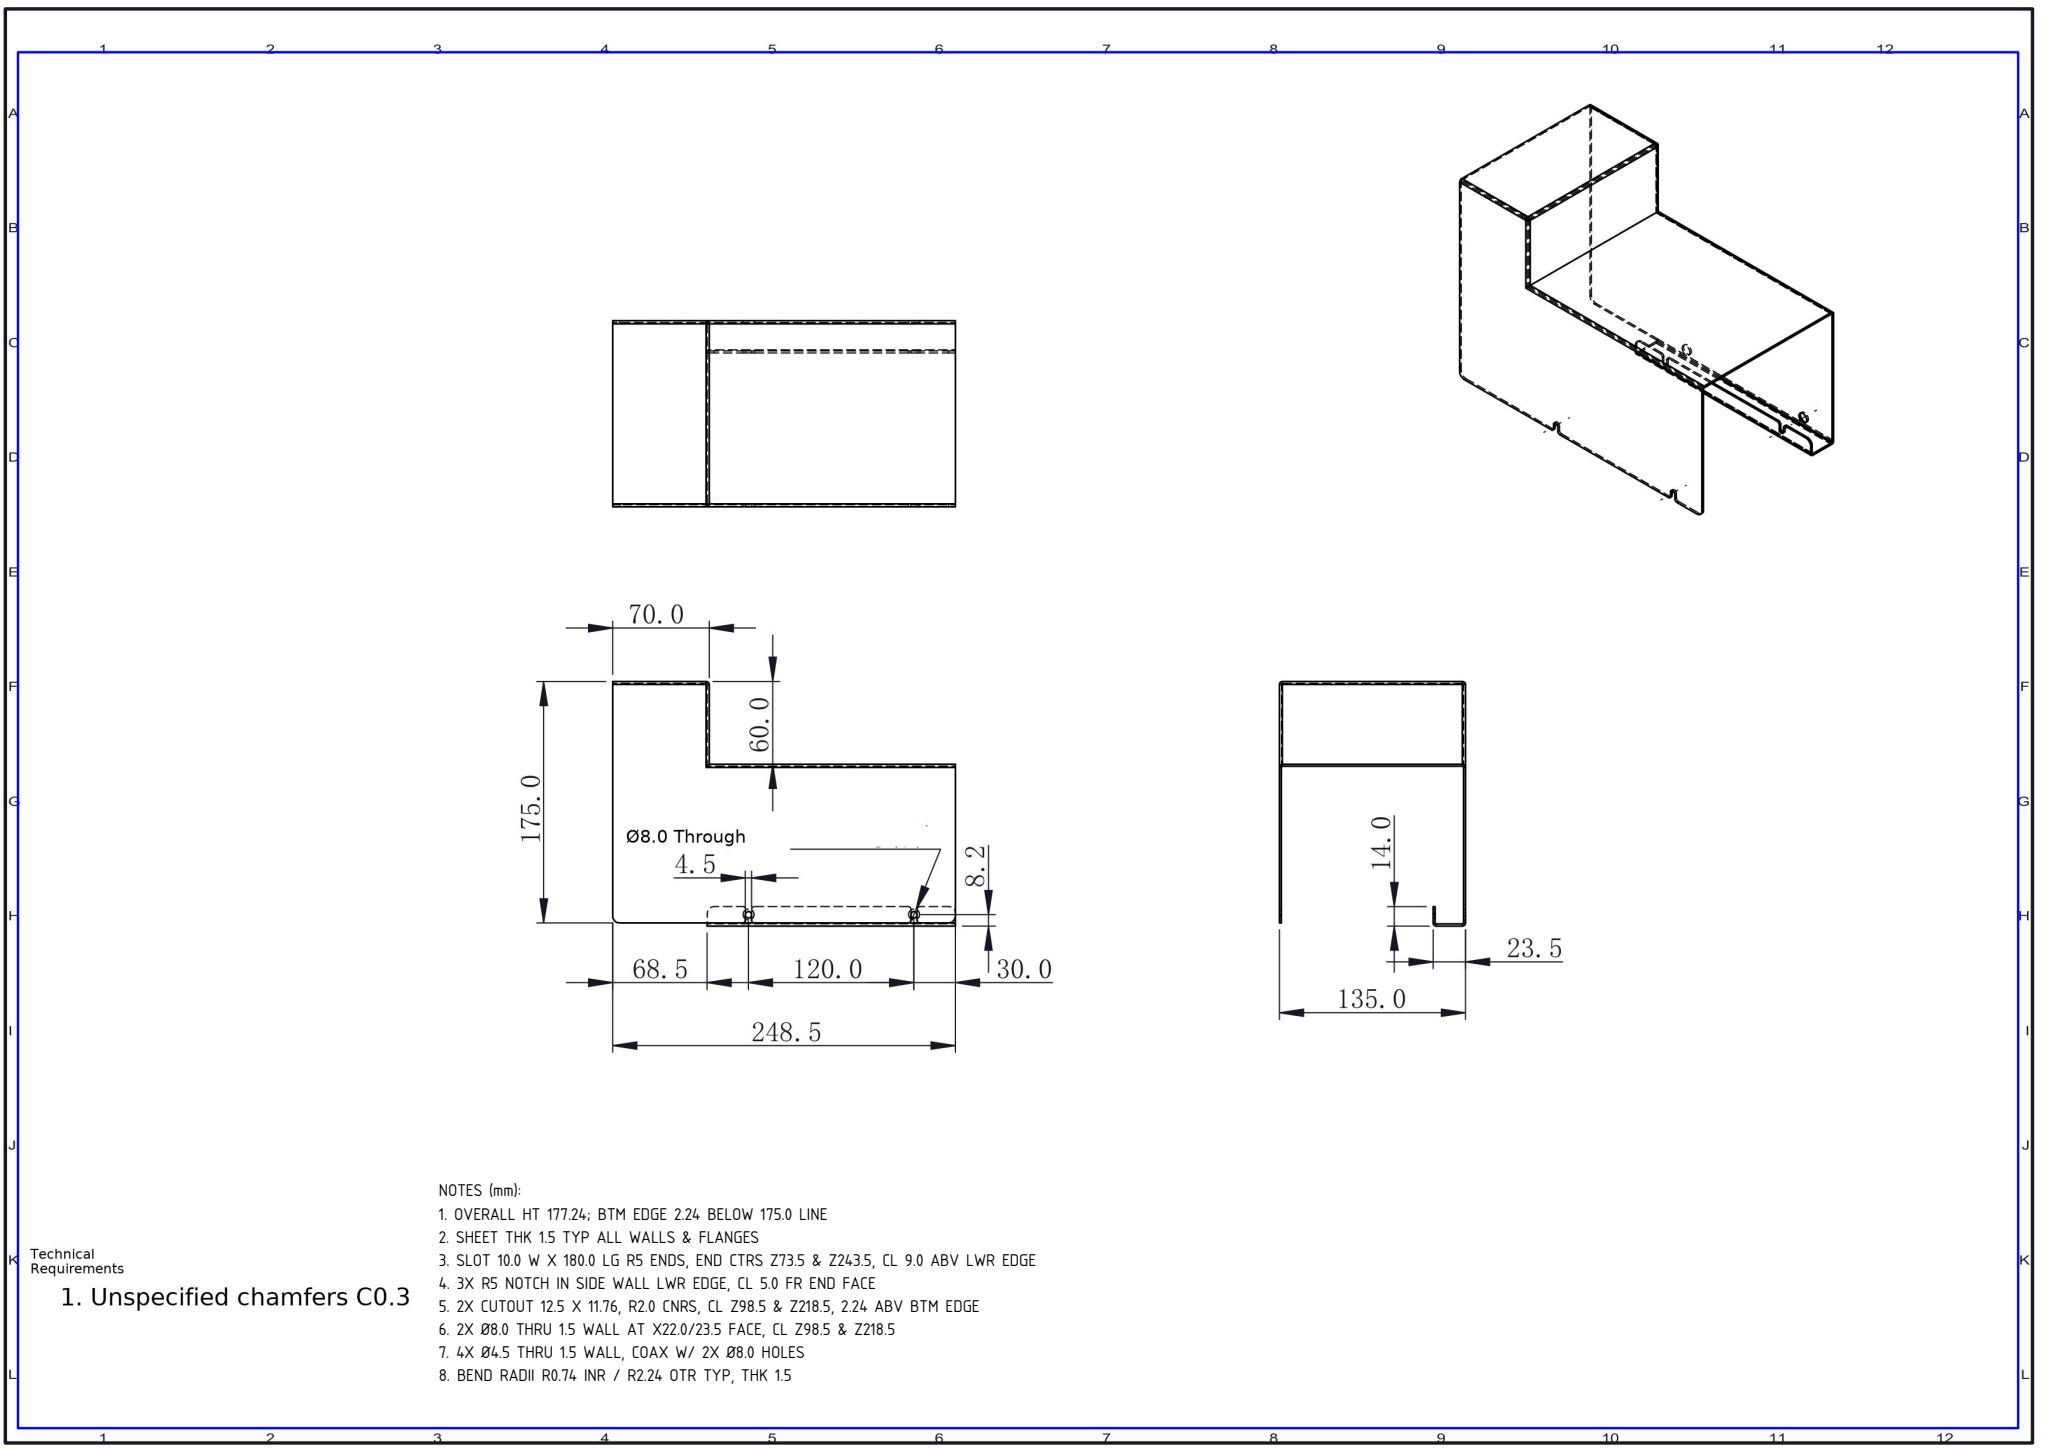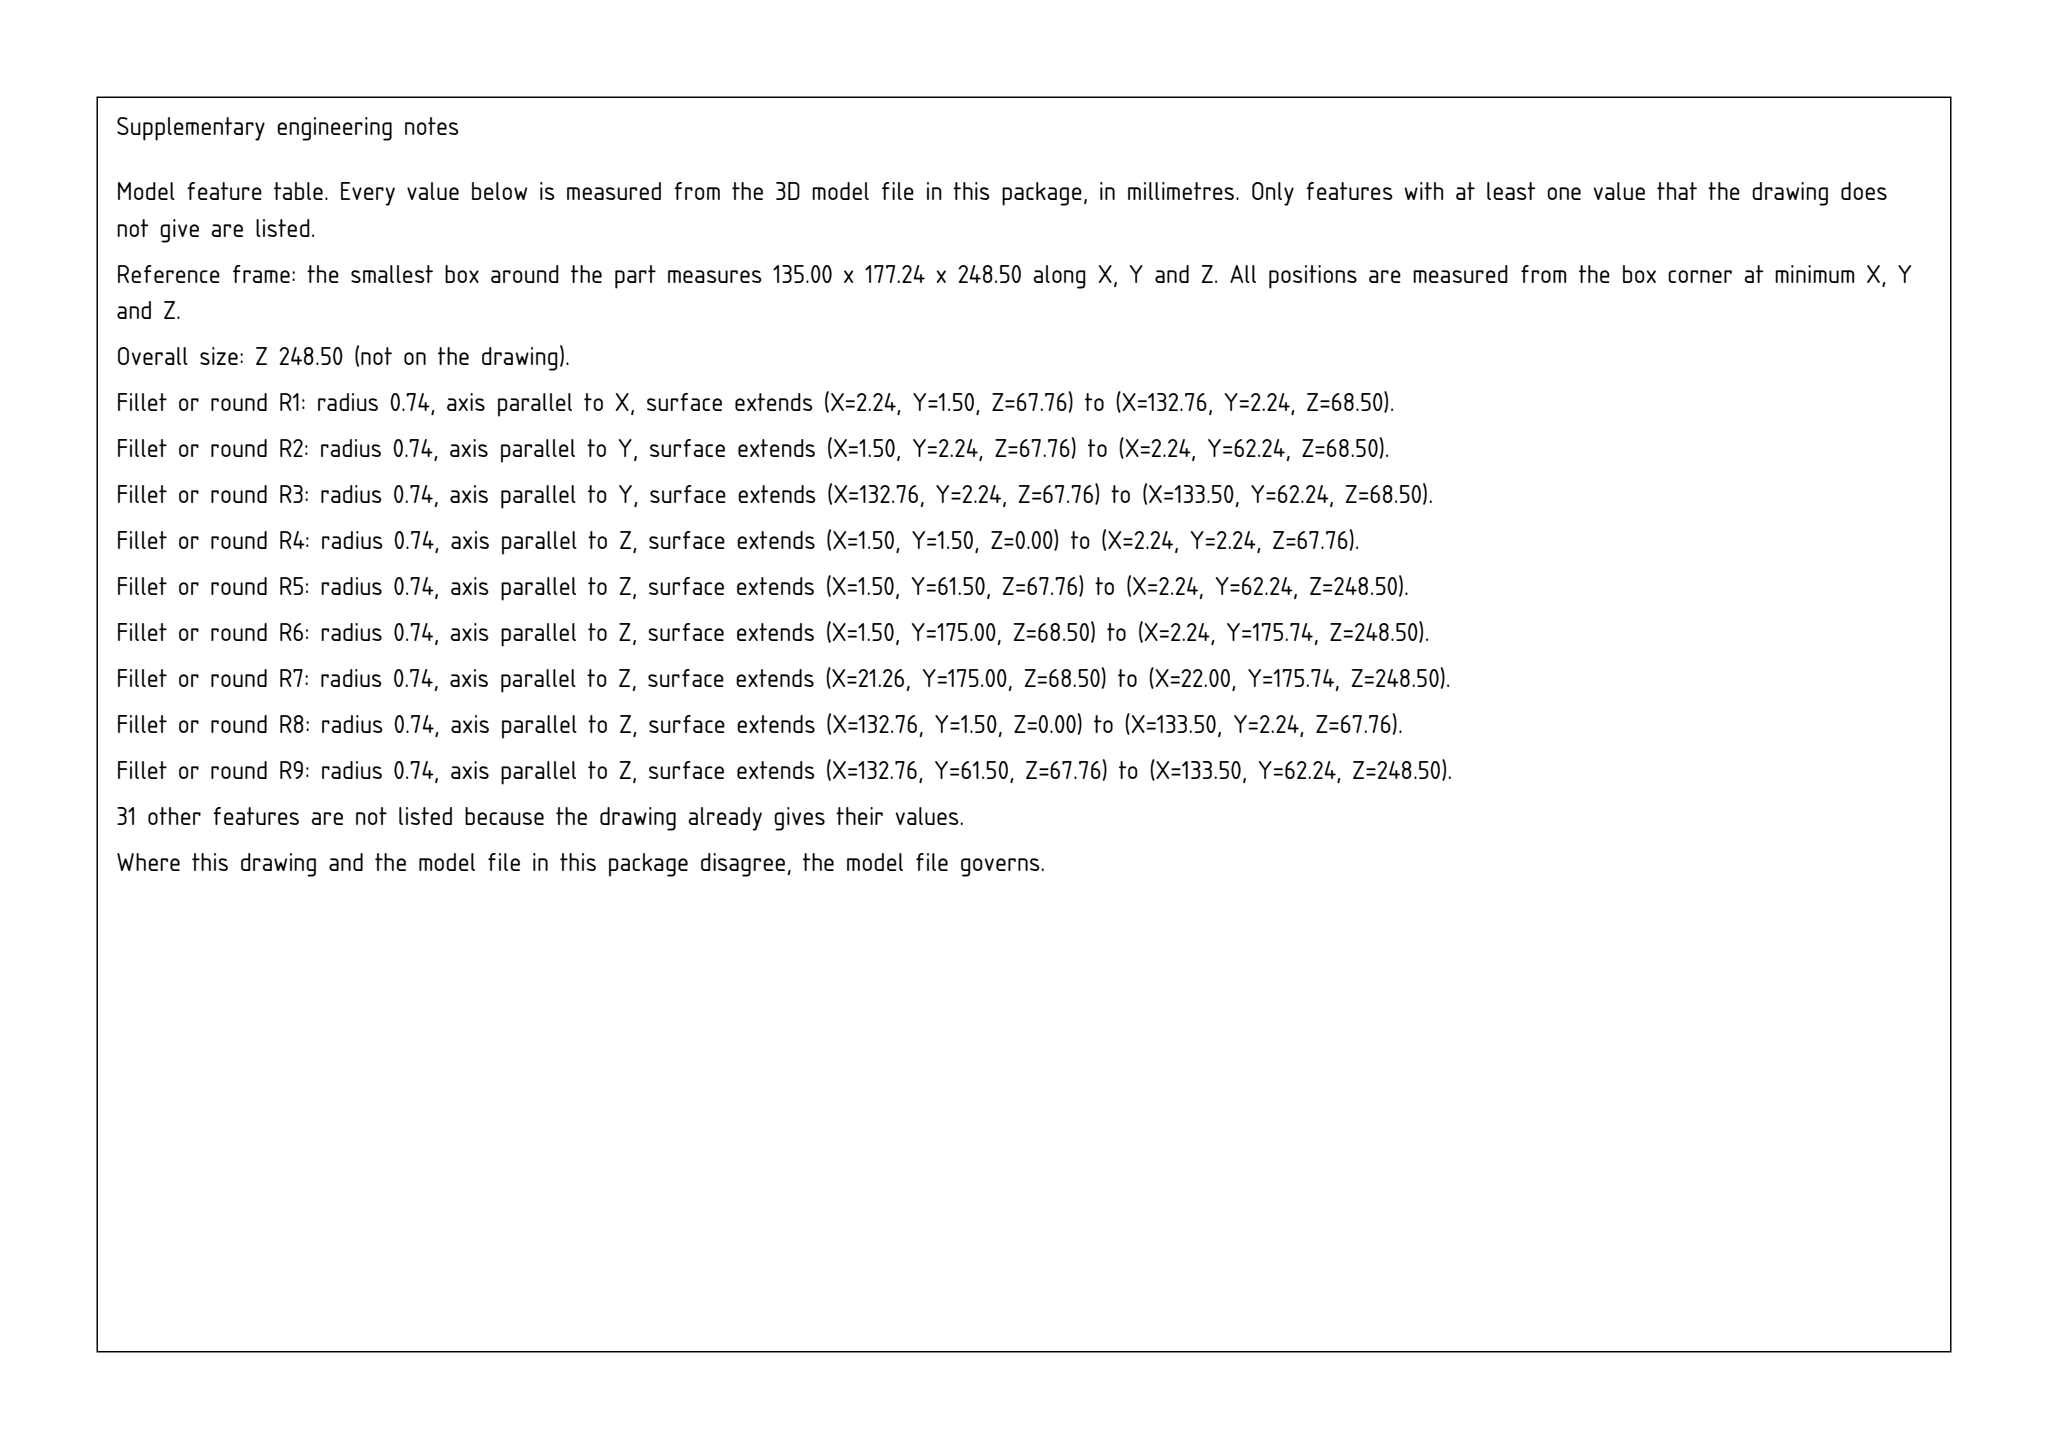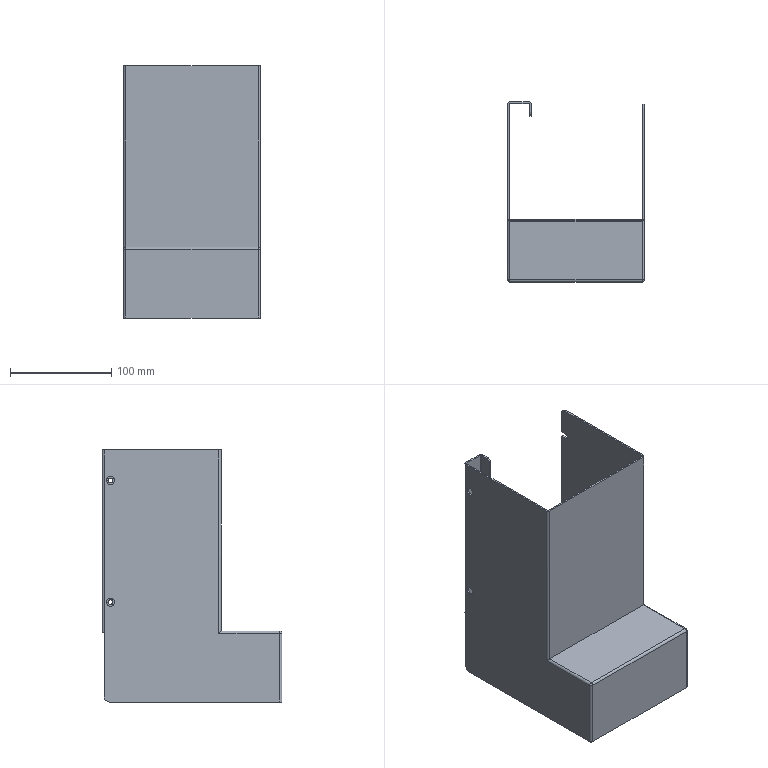Part | SolidWorks | mm | 1 solid | 88 faces | box 135 x 177.24 x 248.5 mm | volume 167859 mm3 | plane 43 | cylinder 41 | sphere 4 | commonest cylinder face diameters 4 x8 4.5 x6 10 x5 1.48 x5 4.48 x5 8 x4 4.473 x4 1.473 x4
Drawing notes:
OVERALL HT 177.24; BTM EDGE 2.24 BELOW 175.0 LINE | from the solid: bbox Y=177.237; y-planes 175.0, 175.74, 177.24 (177.24-175.0=2.24)
SHEET THK 1.5 TYP ALL WALLS & FLANGES | from the solid: Face pairs x=0.0/1.5, 22.0/23.5, 133.5/135.0 and y=0.0/1.5, 175.74/177.24
SLOT 10.0 W X 180.0 LG R5 ENDS, END CTRS Z73.5 & Z243.5, CL 9.0 ABV LWR EDGE | from the solid: Ø10 cyls axis x len 1.5 at (y168.24,z73.5)&(y168.24,z243.5); 243.5-73.5=170.0; z planes 68.5 & 248.5; 177.24-168.24=9.0
3X R5 NOTCH IN SIDE WALL LWR EDGE, CL 5.0 FR END FACE | from the solid: Ø10 cyls axis x len 1.5 at (y170.0,z5.0) x2 and (y170.0,z243.5); end faces z=0 and z=248.5
2X CUTOUT 12.5 X 11.76, R2.0 CNRS, CL Z98.5 & Z218.5, 2.24 ABV BTM EDGE | from the solid: Ø4.0 corner cyls at z=94.25/102.75 & 214.25/222.75, y=165.24/173.0; z planes 96.25/100.75/216.25/220.75; y 163.24 to 175.0
2X Ø8.0 THRU 1.5 WALL AT X22.0/23.5 FACE, CL Z98.5 & Z218.5 | from the solid: Ø8.0 cyls axis x len 1.5 at (y169.0,z98.5)&(y169.0,z218.5); x planes 22.0/23.5
4X Ø4.5 THRU 1.5 WALL, COAX W/ 2X Ø8.0 HOLES | from the solid: Ø4.5 cyls axis x len 1.5 at (y169.0/169.24, z98.5 & z218.5) coaxial with Ø8.0 cyls
BEND RADII R0.74 INR / R2.24 OTR TYP, THK 1.5 | from the solid: Bend cyls dia 1.473/1.48 (R0.74) and 4.473/4.48 (R2.24); wall planes 1.5 apart